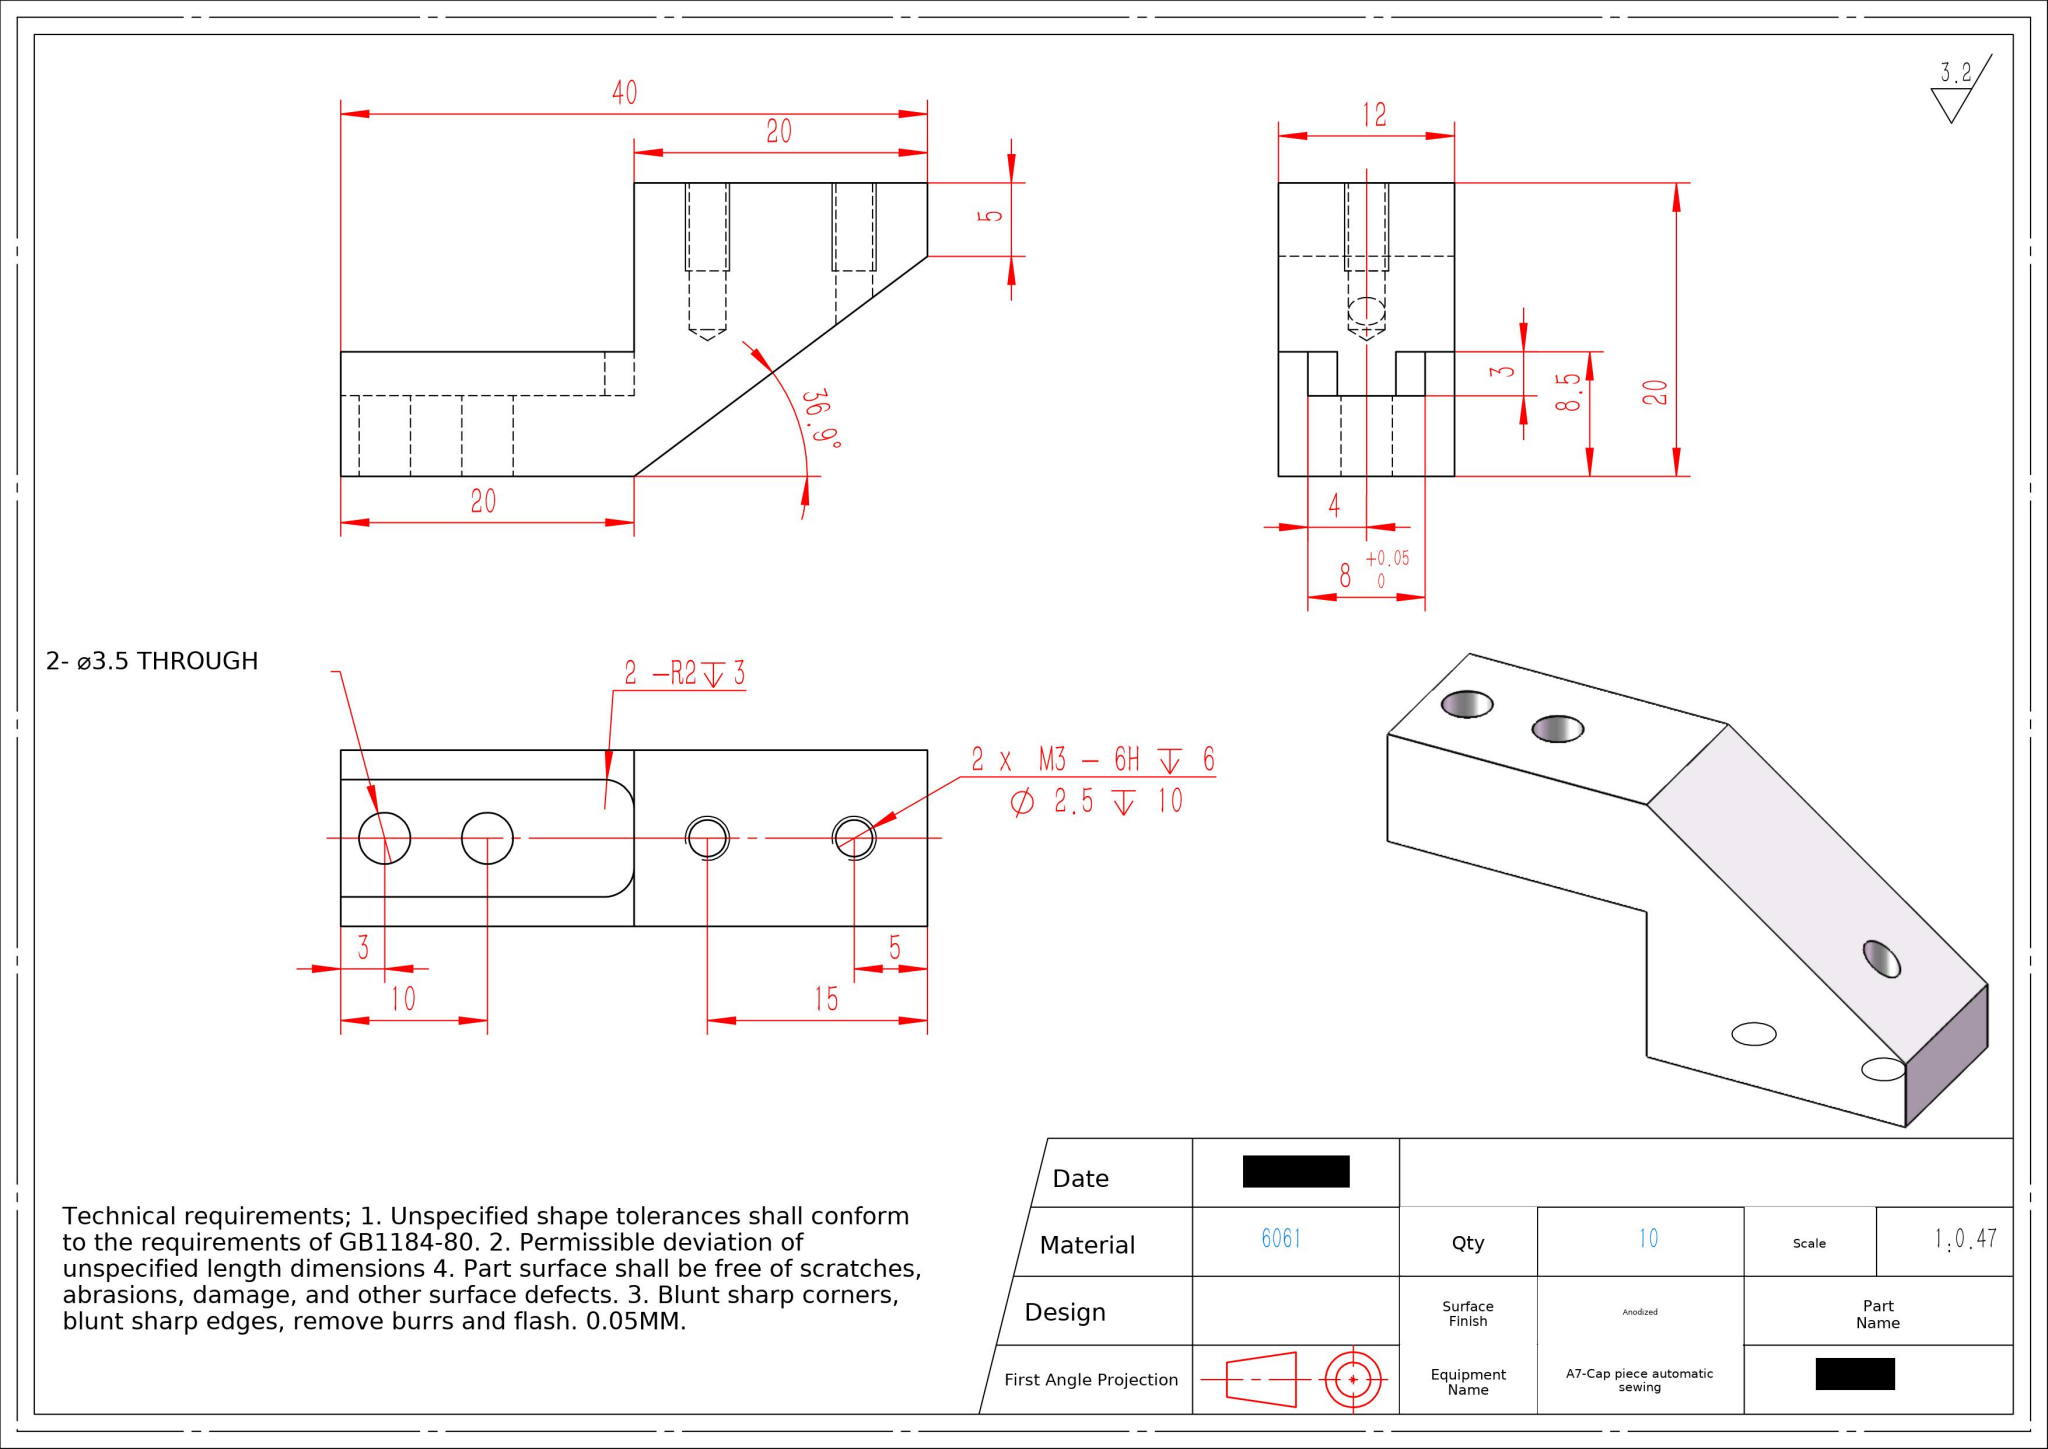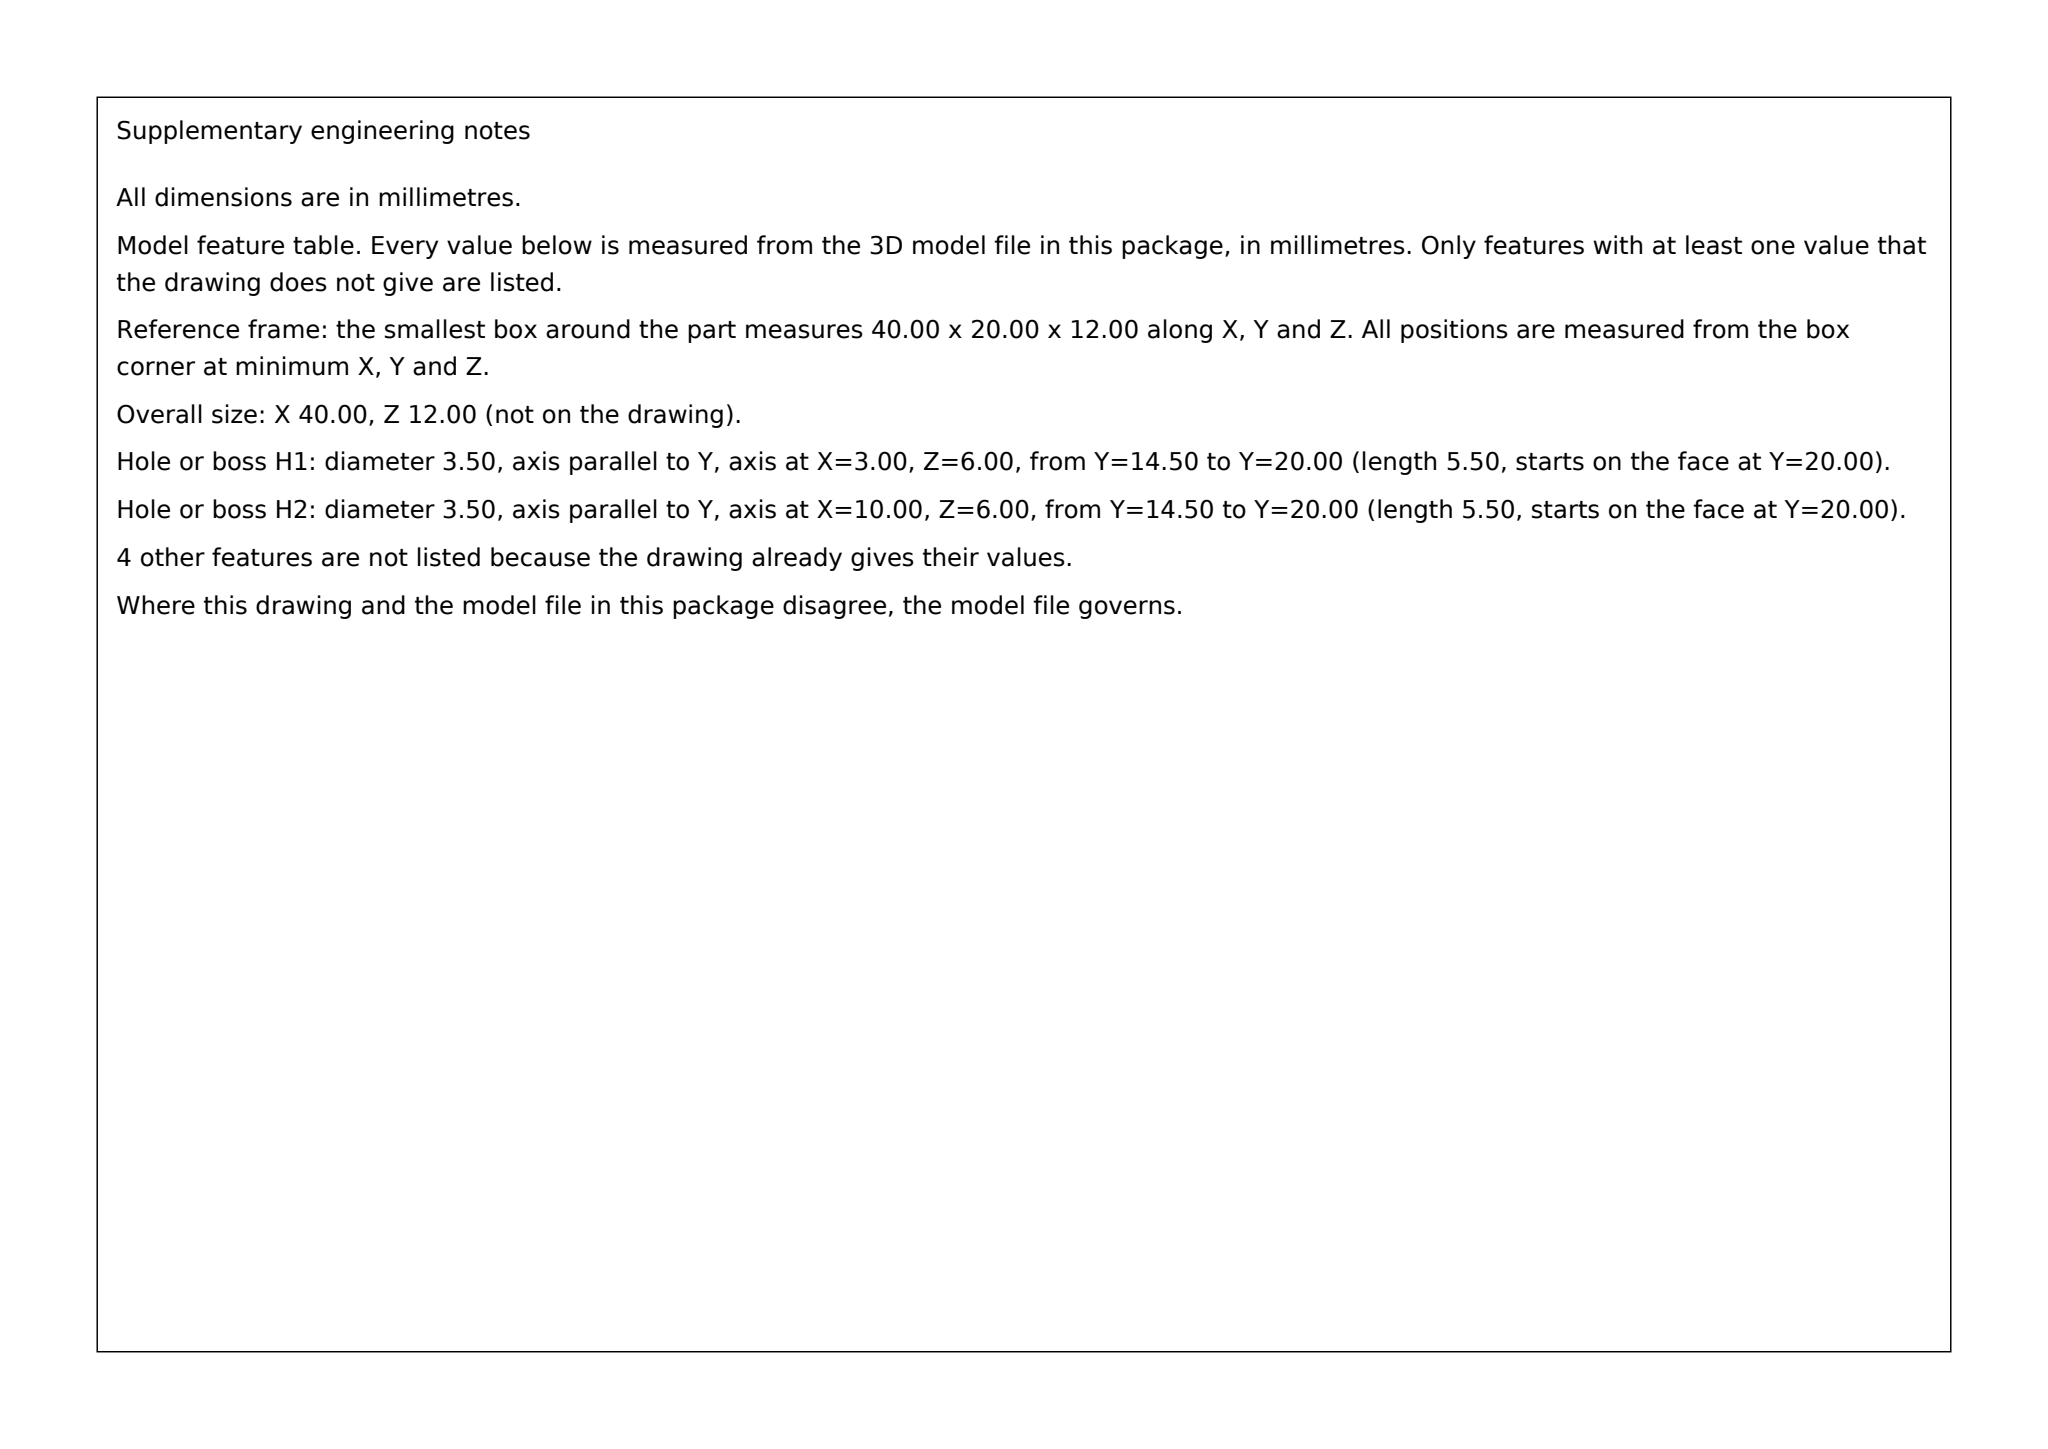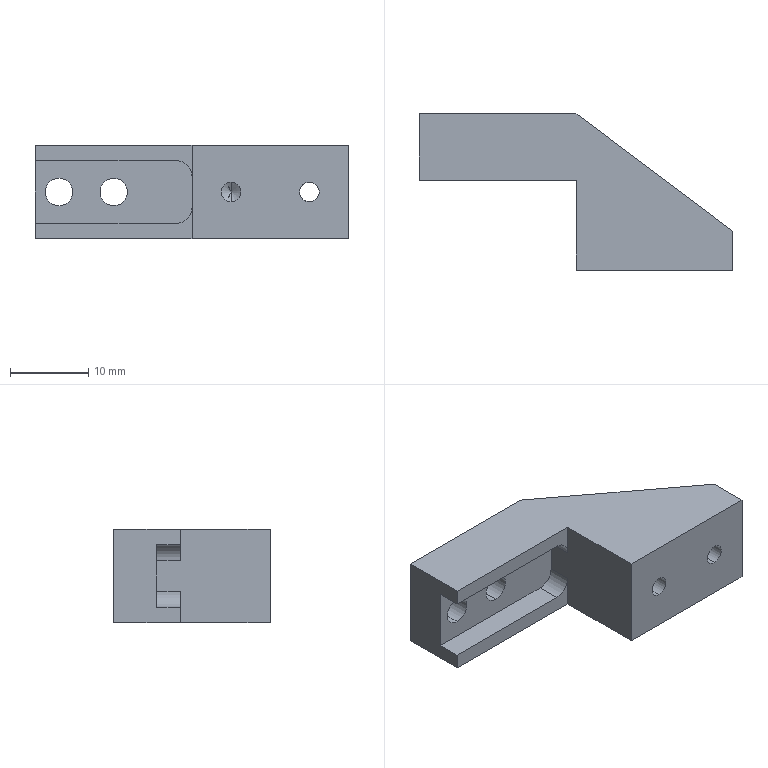Part | SolidWorks | mm | material 6061 | 1 solid | 25 faces | box 40 x 20 x 12 mm | volume 4366 mm3 | plane 13 | cylinder 10 | cone 2 | commonest cylinder face diameters 2.5 x4 3.5 x4 4 x2
build123d program:
from build123d import *

# Parameters (mm, degrees)
SKETCH1_W           = 40
SKETCH1_H           = 12
BOSS_EXTRUDE1_DEPTH = 20
SKETCH2_W           = 20
SKETCH2_H           = 11.5
CUT_EXTRUDE1_DEPTH  = 31.725
SKETCH3_W           = 20
SKETCH3_H           = 8
CUT_EXTRUDE2_DEPTH  = 3
SKETCH4_R           = 1.75
CUT_EXTRUDE3_DEPTH  = 29.914
FILLET1_R           = 2
LPATTERN1_COUNT     = 2
LPATTERN1_PITCH     = 10
CUT_EXTRUDE4_DEPTH  = 31.725


with BuildPart() as part:
    # Sketch1 → Boss-Extrude1 (new body)
    with BuildSketch(Plane(origin=(0, 0, 0), x_dir=(1, 0, 0), z_dir=(0, 1, 0))):
        Rectangle(SKETCH1_W, SKETCH1_H)
    extrude(amount=BOSS_EXTRUDE1_DEPTH)

    # Sketch2 → Cut-Extrude1 (cut, through all)
    with BuildSketch(Plane.XY.offset(6)):
        with Locations((-10, 5.75)):
            Rectangle(SKETCH2_W, SKETCH2_H)
    extrude(amount=-CUT_EXTRUDE1_DEPTH, mode=Mode.SUBTRACT)

    # Sketch3 → Cut-Extrude2 (cut)
    with BuildSketch(Plane(origin=(0, 11.5, 0), x_dir=(-1, 0, 0), z_dir=(0, -1, 0))):
        with Locations((10, 0)):
            Rectangle(SKETCH3_W, SKETCH3_H)
    extrude(amount=-CUT_EXTRUDE2_DEPTH, mode=Mode.SUBTRACT)

    # Sketch4 → Cut-Extrude3 (cut, through all)
    with BuildSketch(Plane(origin=(0, 20, 0), x_dir=(1, 0, 0), z_dir=(0, 1, 0))):
        with Locations(Location((-17, 0, 0), (0, 0, 270))):
            Circle(SKETCH4_R)
        with Locations(Location((-10, 0, 0), (0, 0, 270))):
            Circle(SKETCH4_R)
    extrude(amount=-CUT_EXTRUDE3_DEPTH, mode=Mode.SUBTRACT)

    # Fillet1
    fillet1_edges = [part.edges().sort_by_distance(p)[0] for p in [
        (0, 13, 4),
        (0, 13, -4),
    ]]
    fillet(fillet1_edges, radius=FILLET1_R)

    # Sketch5 → M3 Tapped Hole1 (revolve, cut)
    with BuildSketch(Plane(origin=(5, 0, 0), x_dir=(0, 0, -1), z_dir=(1, 0, 0))):
        Polygon((0, 0), (0, 10.751), (1.25, 10), (1.25, 0), align=None)
    m3_tapped_hole1 = revolve(axis=Axis((5, -6.35, 0), (0, 1, 0)), mode=Mode.SUBTRACT)

    # LPattern1: M3 Tapped Hole1 ×2
    with Locations(*[(i * LPATTERN1_PITCH, 0, 0) for i in range(1, LPATTERN1_COUNT)]):
        add(m3_tapped_hole1, mode=Mode.SUBTRACT)

    # Sketch6 → Cut-Extrude4 (cut, through all)
    with BuildSketch(Plane.XY.offset(6)):
        Polygon((20, 5), (0, 20), (20, 20), align=None)
    extrude(amount=-CUT_EXTRUDE4_DEPTH, mode=Mode.SUBTRACT)


solid = part.part
STEP:
#1=CARTESIAN_POINT('',(15.,8.75,-1.25));
#2=VERTEX_POINT('',#1);
#3=CARTESIAN_POINT('',(15.,8.75,1.25));
#4=VERTEX_POINT('',#3);
#5=CARTESIAN_POINT('',(15.,8.75,-1.25));
#6=CARTESIAN_POINT('',(12.5,10.625,-1.25));
#7=CARTESIAN_POINT('',(12.5,10.625,1.25));
#8=CARTESIAN_POINT('',(15.,8.75,1.25));
#9=(BOUNDED_CURVE()B_SPLINE_CURVE(3,(#5,#6,#7,#8),.UNSPECIFIED.,.F.,.T.)B_SPLINE_CURVE_WITH_KNOTS((4,4),(1.571,4.712),.UNSPECIFIED.)CURVE()GEOMETRIC_REPRESENTATION_ITEM()RATIONAL_B_SPLINE_CURVE((1.,0.3333,0.3333,1.))REPRESENTATION_ITEM(''));
#10=EDGE_CURVE('',#2,#4,#9,.T.);
#11=ORIENTED_EDGE('',*,*,#10,.T.);
#12=CARTESIAN_POINT('',(15.,-0.,1.25));
#13=VERTEX_POINT('',#12);
#14=CARTESIAN_POINT('',(15.,0.,1.25));
#15=DIRECTION('',(0.,-1.,0.));
#16=VECTOR('',#15,1000.);
#17=LINE('',#14,#16);
#18=EDGE_CURVE('',#4,#13,#17,.T.);
#19=ORIENTED_EDGE('',*,*,#18,.T.);
#20=CARTESIAN_POINT('',(15.,-0.,-1.25));
#21=VERTEX_POINT('',#20);
#22=CARTESIAN_POINT('',(15.,-0.,0.));
#23=DIRECTION('',(0.,-1.,0.));
#24=DIRECTION('',(0.,0.,-1.));
#25=AXIS2_PLACEMENT_3D('',#22,#23,#24);
#26=CIRCLE('',#25,1.25);
#27=EDGE_CURVE('',#13,#21,#26,.T.);
#28=ORIENTED_EDGE('',*,*,#27,.T.);
#29=CARTESIAN_POINT('',(15.,0.,-1.25));
#30=DIRECTION('',(0.,-1.,0.));
#31=VECTOR('',#30,1000.);
#32=LINE('',#29,#31);
#33=EDGE_CURVE('',#2,#21,#32,.T.);
#34=ORIENTED_EDGE('',*,*,#33,.F.);
#35=EDGE_LOOP('',(#11,#19,#28,#34));
#36=FACE_OUTER_BOUND('',#35,.T.);
#37=CARTESIAN_POINT('',(15.,0.,0.));
#38=DIRECTION('',(0.,-1.,0.));
#39=DIRECTION('',(0.,0.,-1.));
#40=AXIS2_PLACEMENT_3D('',#37,#38,#39);
#41=CYLINDRICAL_SURFACE('',#40,1.25);
#42=ADVANCED_FACE('',(#36),#41,.F.);
#43=CARTESIAN_POINT('',(5.,10.,1.25));
#44=VERTEX_POINT('',#43);
#45=CARTESIAN_POINT('',(5.,10.,-1.25));
#46=VERTEX_POINT('',#45);
#47=CARTESIAN_POINT('',(5.,10.,0.));
#48=DIRECTION('',(0.,-1.,0.));
#49=DIRECTION('',(0.,0.,-1.));
#50=AXIS2_PLACEMENT_3D('',#47,#48,#49);
#51=CIRCLE('',#50,1.25);
#52=EDGE_CURVE('',#44,#46,#51,.T.);
#53=ORIENTED_EDGE('',*,*,#52,.F.);
#54=CARTESIAN_POINT('',(5.,-0.,1.25));
#55=VERTEX_POINT('',#54);
#56=CARTESIAN_POINT('',(5.,0.,1.25));
#57=DIRECTION('',(0.,-1.,0.));
#58=VECTOR('',#57,1000.);
#59=LINE('',#56,#58);
#60=EDGE_CURVE('',#44,#55,#59,.T.);
#61=ORIENTED_EDGE('',*,*,#60,.T.);
#62=CARTESIAN_POINT('',(5.,-0.,-1.25));
#63=VERTEX_POINT('',#62);
#64=CARTESIAN_POINT('',(5.,-0.,0.));
#65=DIRECTION('',(0.,-1.,0.));
#66=DIRECTION('',(0.,0.,-1.));
#67=AXIS2_PLACEMENT_3D('',#64,#65,#66);
#68=CIRCLE('',#67,1.25);
#69=EDGE_CURVE('',#55,#63,#68,.T.);
#70=ORIENTED_EDGE('',*,*,#69,.T.);
#71=CARTESIAN_POINT('',(5.,0.,-1.25));
#72=DIRECTION('',(0.,-1.,0.));
#73=VECTOR('',#72,1000.);
#74=LINE('',#71,#73);
#75=EDGE_CURVE('',#46,#63,#74,.T.);
#76=ORIENTED_EDGE('',*,*,#75,.F.);
#77=EDGE_LOOP('',(#53,#61,#70,#76));
#78=FACE_OUTER_BOUND('',#77,.T.);
#79=CARTESIAN_POINT('',(5.,0.,0.));
#80=DIRECTION('',(0.,-1.,0.));
#81=DIRECTION('',(0.,0.,-1.));
#82=AXIS2_PLACEMENT_3D('',#79,#80,#81);
#83=CYLINDRICAL_SURFACE('',#82,1.25);
#84=ADVANCED_FACE('',(#78),#83,.F.);
#85=CARTESIAN_POINT('',(5.,10.751,0.));
#86=VERTEX_POINT('',#85);
#87=CARTESIAN_POINT('',(5.,10.,-1.25));
#88=DIRECTION('',(0.,-0.515,-0.8572));
#89=VECTOR('',#88,1000.);
#90=LINE('',#87,#89);
#91=EDGE_CURVE('',#86,#46,#90,.T.);
#92=ORIENTED_EDGE('',*,*,#91,.F.);
#93=CARTESIAN_POINT('',(5.,10.,1.25));
#94=DIRECTION('',(0.,-0.515,0.8572));
#95=VECTOR('',#94,1000.);
#96=LINE('',#93,#95);
#97=EDGE_CURVE('',#86,#44,#96,.T.);
#98=ORIENTED_EDGE('',*,*,#97,.T.);
#99=ORIENTED_EDGE('',*,*,#52,.T.);
#100=EDGE_LOOP('',(#92,#98,#99));
#101=FACE_OUTER_BOUND('',#100,.T.);
#102=CARTESIAN_POINT('',(5.,10.,0.));
#103=DIRECTION('',(0.,-1.,0.));
#104=DIRECTION('',(0.,0.,-1.));
#105=AXIS2_PLACEMENT_3D('',#102,#103,#104);
#106=CONICAL_SURFACE('',#105,1.25,1.03);
#107=ADVANCED_FACE('',(#101),#106,.F.);
#108=CARTESIAN_POINT('',(-17.,14.5,1.75));
#109=VERTEX_POINT('',#108);
#110=CARTESIAN_POINT('',(-17.,14.5,-1.75));
#111=VERTEX_POINT('',#110);
#112=CARTESIAN_POINT('',(-17.,14.5,0.));
#113=DIRECTION('',(0.,-1.,0.));
#114=DIRECTION('',(0.,0.,-1.));
#115=AXIS2_PLACEMENT_3D('',#112,#113,#114);
#116=CIRCLE('',#115,1.75);
#117=EDGE_CURVE('',#109,#111,#116,.T.);
#118=ORIENTED_EDGE('',*,*,#117,.T.);
#119=CARTESIAN_POINT('',(-17.,20.,-1.75));
#120=VERTEX_POINT('',#119);
#121=CARTESIAN_POINT('',(-17.,0.,-1.75));
#122=DIRECTION('',(0.,1.,0.));
#123=VECTOR('',#122,1000.);
#124=LINE('',#121,#123);
#125=EDGE_CURVE('',#111,#120,#124,.T.);
#126=ORIENTED_EDGE('',*,*,#125,.T.);
#127=CARTESIAN_POINT('',(-17.,20.,1.75));
#128=VERTEX_POINT('',#127);
#129=CARTESIAN_POINT('',(-17.,20.,0.));
#130=DIRECTION('',(0.,1.,0.));
#131=DIRECTION('',(0.,0.,1.));
#132=AXIS2_PLACEMENT_3D('',#129,#130,#131);
#133=CIRCLE('',#132,1.75);
#134=EDGE_CURVE('',#120,#128,#133,.T.);
#135=ORIENTED_EDGE('',*,*,#134,.T.);
#136=CARTESIAN_POINT('',(-17.,0.,1.75));
#137=DIRECTION('',(0.,1.,0.));
#138=VECTOR('',#137,1000.);
#139=LINE('',#136,#138);
#140=EDGE_CURVE('',#109,#128,#139,.T.);
#141=ORIENTED_EDGE('',*,*,#140,.F.);
#142=EDGE_LOOP('',(#118,#126,#135,#141));
#143=FACE_OUTER_BOUND('',#142,.T.);
#144=CARTESIAN_POINT('',(-17.,0.,0.));
#145=DIRECTION('',(0.,1.,0.));
#146=DIRECTION('',(0.,0.,1.));
#147=AXIS2_PLACEMENT_3D('',#144,#145,#146);
#148=CYLINDRICAL_SURFACE('',#147,1.75);
#149=ADVANCED_FACE('',(#143),#148,.F.);
#150=CARTESIAN_POINT('',(-10.,14.5,1.75));
#151=VERTEX_POINT('',#150);
#152=CARTESIAN_POINT('',(-10.,14.5,-1.75));
#153=VERTEX_POINT('',#152);
#154=CARTESIAN_POINT('',(-10.,14.5,0.));
#155=DIRECTION('',(0.,-1.,0.));
#156=DIRECTION('',(0.,0.,-1.));
#157=AXIS2_PLACEMENT_3D('',#154,#155,#156);
#158=CIRCLE('',#157,1.75);
#159=EDGE_CURVE('',#151,#153,#158,.T.);
#160=ORIENTED_EDGE('',*,*,#159,.T.);
#161=CARTESIAN_POINT('',(-10.,20.,-1.75));
#162=VERTEX_POINT('',#161);
#163=CARTESIAN_POINT('',(-10.,0.,-1.75));
#164=DIRECTION('',(0.,1.,0.));
#165=VECTOR('',#164,1000.);
#166=LINE('',#163,#165);
#167=EDGE_CURVE('',#153,#162,#166,.T.);
#168=ORIENTED_EDGE('',*,*,#167,.T.);
#169=CARTESIAN_POINT('',(-10.,20.,1.75));
#170=VERTEX_POINT('',#169);
#171=CARTESIAN_POINT('',(-10.,20.,0.));
#172=DIRECTION('',(0.,1.,0.));
#173=DIRECTION('',(0.,0.,1.));
#174=AXIS2_PLACEMENT_3D('',#171,#172,#173);
#175=CIRCLE('',#174,1.75);
#176=EDGE_CURVE('',#162,#170,#175,.T.);
#177=ORIENTED_EDGE('',*,*,#176,.T.);
#178=CARTESIAN_POINT('',(-10.,0.,1.75));
#179=DIRECTION('',(0.,1.,0.));
#180=VECTOR('',#179,1000.);
#181=LINE('',#178,#180);
#182=EDGE_CURVE('',#151,#170,#181,.T.);
#183=ORIENTED_EDGE('',*,*,#182,.F.);
#184=EDGE_LOOP('',(#160,#168,#177,#183));
#185=FACE_OUTER_BOUND('',#184,.T.);
#186=CARTESIAN_POINT('',(-10.,0.,0.));
#187=DIRECTION('',(0.,1.,0.));
#188=DIRECTION('',(0.,0.,1.));
#189=AXIS2_PLACEMENT_3D('',#186,#187,#188);
#190=CYLINDRICAL_SURFACE('',#189,1.75);
#191=ADVANCED_FACE('',(#185),#190,.F.);
#192=CARTESIAN_POINT('',(0.,11.5,-6.));
#193=VERTEX_POINT('',#192);
#194=CARTESIAN_POINT('',(0.,11.5,-2.));
#195=VERTEX_POINT('',#194);
#196=CARTESIAN_POINT('',(0.,11.5,-6.));
#197=DIRECTION('',(0.,0.,1.));
#198=VECTOR('',#197,1000.);
#199=LINE('',#196,#198);
#200=EDGE_CURVE('',#193,#195,#199,.T.);
#201=ORIENTED_EDGE('',*,*,#200,.T.);
#202=CARTESIAN_POINT('',(-2.,11.5,-4.));
#203=VERTEX_POINT('',#202);
#204=CARTESIAN_POINT('',(-2.,11.5,-2.));
#205=DIRECTION('',(0.,1.,0.));
#206=DIRECTION('',(0.,0.,1.));
#207=AXIS2_PLACEMENT_3D('',#204,#205,#206);
#208=CIRCLE('',#207,2.);
#209=EDGE_CURVE('',#195,#203,#208,.T.);
#210=ORIENTED_EDGE('',*,*,#209,.T.);
#211=CARTESIAN_POINT('',(-20.,11.5,-4.));
#212=VERTEX_POINT('',#211);
#213=CARTESIAN_POINT('',(-20.,11.5,-4.));
#214=DIRECTION('',(1.,0.,0.));
#215=VECTOR('',#214,1000.);
#216=LINE('',#213,#215);
#217=EDGE_CURVE('',#212,#203,#216,.T.);
#218=ORIENTED_EDGE('',*,*,#217,.F.);
#219=CARTESIAN_POINT('',(-20.,11.5,-6.));
#220=VERTEX_POINT('',#219);
#221=CARTESIAN_POINT('',(-20.,11.5,-6.));
#222=DIRECTION('',(0.,0.,1.));
#223=VECTOR('',#222,1000.);
#224=LINE('',#221,#223);
#225=EDGE_CURVE('',#220,#212,#224,.T.);
#226=ORIENTED_EDGE('',*,*,#225,.F.);
#227=CARTESIAN_POINT('',(-20.,11.5,-6.));
#228=DIRECTION('',(-1.,0.,0.));
#229=VECTOR('',#228,1000.);
#230=LINE('',#227,#229);
#231=EDGE_CURVE('',#193,#220,#230,.T.);
#232=ORIENTED_EDGE('',*,*,#231,.F.);
#233=EDGE_LOOP('',(#201,#210,#218,#226,#232));
#234=FACE_OUTER_BOUND('',#233,.T.);
#235=CARTESIAN_POINT('',(-20.,11.5,-6.));
#236=DIRECTION('',(0.,1.,0.));
#237=DIRECTION('',(0.,0.,1.));
#238=AXIS2_PLACEMENT_3D('',#235,#236,#237);
#239=PLANE('',#238);
#240=ADVANCED_FACE('',(#234),#239,.F.);
#241=CARTESIAN_POINT('',(20.,5.,-6.));
#242=VERTEX_POINT('',#241);
#243=CARTESIAN_POINT('',(20.,0.,-6.));
#244=VERTEX_POINT('',#243);
#245=CARTESIAN_POINT('',(20.,20.,-6.));
#246=DIRECTION('',(0.,-1.,0.));
#247=VECTOR('',#246,1000.);
#248=LINE('',#245,#247);
#249=EDGE_CURVE('',#242,#244,#248,.T.);
#250=ORIENTED_EDGE('',*,*,#249,.F.);
#251=CARTESIAN_POINT('',(20.,5.,6.));
#252=VERTEX_POINT('',#251);
#253=CARTESIAN_POINT('',(20.,5.,-6.));
#254=DIRECTION('',(0.,0.,1.));
#255=VECTOR('',#254,1000.);
#256=LINE('',#253,#255);
#257=EDGE_CURVE('',#242,#252,#256,.T.);
#258=ORIENTED_EDGE('',*,*,#257,.T.);
#259=CARTESIAN_POINT('',(20.,0.,6.));
#260=VERTEX_POINT('',#259);
#261=CARTESIAN_POINT('',(20.,20.,6.));
#262=DIRECTION('',(0.,-1.,0.));
#263=VECTOR('',#262,1000.);
#264=LINE('',#261,#263);
#265=EDGE_CURVE('',#252,#260,#264,.T.);
#266=ORIENTED_EDGE('',*,*,#265,.T.);
#267=CARTESIAN_POINT('',(20.,0.,-6.));
#268=DIRECTION('',(0.,0.,-1.));
#269=VECTOR('',#268,1000.);
#270=LINE('',#267,#269);
#271=EDGE_CURVE('',#260,#244,#270,.T.);
#272=ORIENTED_EDGE('',*,*,#271,.T.);
#273=EDGE_LOOP('',(#250,#258,#266,#272));
#274=FACE_OUTER_BOUND('',#273,.T.);
#275=CARTESIAN_POINT('',(20.,20.,-6.));
#276=DIRECTION('',(-1.,0.,0.));
#277=DIRECTION('',(0.,0.,1.));
#278=AXIS2_PLACEMENT_3D('',#275,#276,#277);
#279=PLANE('',#278);
#280=ADVANCED_FACE('',(#274),#279,.F.);
#281=CARTESIAN_POINT('',(-0.,20.,-6.));
#282=VERTEX_POINT('',#281);
#283=CARTESIAN_POINT('',(-20.,20.,-6.));
#284=VERTEX_POINT('',#283);
#285=CARTESIAN_POINT('',(-20.,20.,-6.));
#286=DIRECTION('',(-1.,0.,0.));
#287=VECTOR('',#286,1000.);
#288=LINE('',#285,#287);
#289=EDGE_CURVE('',#282,#284,#288,.T.);
#290=ORIENTED_EDGE('',*,*,#289,.F.);
#291=CARTESIAN_POINT('',(20.,5.,-6.));
#292=DIRECTION('',(0.8,-0.6,0.));
#293=VECTOR('',#292,1000.);
#294=LINE('',#291,#293);
#295=EDGE_CURVE('',#282,#242,#294,.T.);
#296=ORIENTED_EDGE('',*,*,#295,.T.);
#297=ORIENTED_EDGE('',*,*,#249,.T.);
#298=CARTESIAN_POINT('',(0.,0.,-6.));
#299=VERTEX_POINT('',#298);
#300=CARTESIAN_POINT('',(-20.,0.,-6.));
#301=DIRECTION('',(-1.,0.,0.));
#302=VECTOR('',#301,1000.);
#303=LINE('',#300,#302);
#304=EDGE_CURVE('',#244,#299,#303,.T.);
#305=ORIENTED_EDGE('',*,*,#304,.T.);
#306=CARTESIAN_POINT('',(0.,0.,-6.));
#307=DIRECTION('',(0.,1.,0.));
#308=VECTOR('',#307,1000.);
#309=LINE('',#306,#308);
#310=EDGE_CURVE('',#299,#193,#309,.T.);
#311=ORIENTED_EDGE('',*,*,#310,.T.);
#312=ORIENTED_EDGE('',*,*,#231,.T.);
#313=CARTESIAN_POINT('',(-20.,20.,-6.));
#314=DIRECTION('',(0.,-1.,0.));
#315=VECTOR('',#314,1000.);
#316=LINE('',#313,#315);
#317=EDGE_CURVE('',#284,#220,#316,.T.);
#318=ORIENTED_EDGE('',*,*,#317,.F.);
#319=EDGE_LOOP('',(#290,#296,#297,#305,#311,#312,#318));
#320=FACE_OUTER_BOUND('',#319,.T.);
#321=CARTESIAN_POINT('',(-20.,20.,-6.));
#322=DIRECTION('',(0.,0.,1.));
#323=DIRECTION('',(1.,0.,0.));
#324=AXIS2_PLACEMENT_3D('',#321,#322,#323);
#325=PLANE('',#324);
#326=ADVANCED_FACE('',(#320),#325,.F.);
#327=ORIENTED_EDGE('',*,*,#225,.T.);
#328=CARTESIAN_POINT('',(-20.,14.5,-4.));
#329=VERTEX_POINT('',#328);
#330=CARTESIAN_POINT('',(-20.,14.5,-4.));
#331=DIRECTION('',(0.,-1.,0.));
#332=VECTOR('',#331,1000.);
#333=LINE('',#330,#332);
#334=EDGE_CURVE('',#329,#212,#333,.T.);
#335=ORIENTED_EDGE('',*,*,#334,.F.);
#336=CARTESIAN_POINT('',(-20.,14.5,4.));
#337=VERTEX_POINT('',#336);
#338=CARTESIAN_POINT('',(-20.,14.5,4.));
#339=DIRECTION('',(0.,0.,-1.));
#340=VECTOR('',#339,1000.);
#341=LINE('',#338,#340);
#342=EDGE_CURVE('',#337,#329,#341,.T.);
#343=ORIENTED_EDGE('',*,*,#342,.F.);
#344=CARTESIAN_POINT('',(-20.,11.5,4.));
#345=VERTEX_POINT('',#344);
#346=CARTESIAN_POINT('',(-20.,14.5,4.));
#347=DIRECTION('',(0.,-1.,0.));
#348=VECTOR('',#347,1000.);
#349=LINE('',#346,#348);
#350=EDGE_CURVE('',#337,#345,#349,.T.);
#351=ORIENTED_EDGE('',*,*,#350,.T.);
#352=CARTESIAN_POINT('',(-20.,11.5,6.));
#353=VERTEX_POINT('',#352);
#354=CARTESIAN_POINT('',(-20.,11.5,-6.));
#355=DIRECTION('',(0.,0.,1.));
#356=VECTOR('',#355,1000.);
#357=LINE('',#354,#356);
#358=EDGE_CURVE('',#345,#353,#357,.T.);
#359=ORIENTED_EDGE('',*,*,#358,.T.);
#360=CARTESIAN_POINT('',(-20.,20.,6.));
#361=VERTEX_POINT('',#360);
#362=CARTESIAN_POINT('',(-20.,20.,6.));
#363=DIRECTION('',(0.,-1.,0.));
#364=VECTOR('',#363,1000.);
#365=LINE('',#362,#364);
#366=EDGE_CURVE('',#361,#353,#365,.T.);
#367=ORIENTED_EDGE('',*,*,#366,.F.);
#368=CARTESIAN_POINT('',(-20.,20.,-6.));
#369=DIRECTION('',(0.,0.,1.));
#370=VECTOR('',#369,1000.);
#371=LINE('',#368,#370);
#372=EDGE_CURVE('',#284,#361,#371,.T.);
#373=ORIENTED_EDGE('',*,*,#372,.F.);
#374=ORIENTED_EDGE('',*,*,#317,.T.);
#375=EDGE_LOOP('',(#327,#335,#343,#351,#359,#367,#373,#374));
#376=FACE_OUTER_BOUND('',#375,.T.);
#377=CARTESIAN_POINT('',(-20.,20.,-6.));
#378=DIRECTION('',(1.,0.,0.));
#379=DIRECTION('',(0.,0.,-1.));
#380=AXIS2_PLACEMENT_3D('',#377,#378,#379);
#381=PLANE('',#380);
#382=ADVANCED_FACE('',(#376),#381,.F.);
#383=ORIENTED_EDGE('',*,*,#265,.F.);
#384=CARTESIAN_POINT('',(-0.,20.,6.));
#385=VERTEX_POINT('',#384);
#386=CARTESIAN_POINT('',(20.,5.,6.));
#387=DIRECTION('',(0.8,-0.6,0.));
#388=VECTOR('',#387,1000.);
#389=LINE('',#386,#388);
#390=EDGE_CURVE('',#385,#252,#389,.T.);
#391=ORIENTED_EDGE('',*,*,#390,.F.);
#392=CARTESIAN_POINT('',(-20.,20.,6.));
#393=DIRECTION('',(1.,0.,0.));
#394=VECTOR('',#393,1000.);
#395=LINE('',#392,#394);
#396=EDGE_CURVE('',#361,#385,#395,.T.);
#397=ORIENTED_EDGE('',*,*,#396,.F.);
#398=ORIENTED_EDGE('',*,*,#366,.T.);
#399=CARTESIAN_POINT('',(0.,11.5,6.));
#400=VERTEX_POINT('',#399);
#401=CARTESIAN_POINT('',(-20.,11.5,6.));
#402=DIRECTION('',(-1.,0.,0.));
#403=VECTOR('',#402,1000.);
#404=LINE('',#401,#403);
#405=EDGE_CURVE('',#400,#353,#404,.T.);
#406=ORIENTED_EDGE('',*,*,#405,.F.);
#407=CARTESIAN_POINT('',(0.,0.,6.));
#408=VERTEX_POINT('',#407);
#409=CARTESIAN_POINT('',(0.,0.,6.));
#410=DIRECTION('',(0.,1.,0.));
#411=VECTOR('',#410,1000.);
#412=LINE('',#409,#411);
#413=EDGE_CURVE('',#408,#400,#412,.T.);
#414=ORIENTED_EDGE('',*,*,#413,.F.);
#415=CARTESIAN_POINT('',(-20.,0.,6.));
#416=DIRECTION('',(1.,0.,0.));
#417=VECTOR('',#416,1000.);
#418=LINE('',#415,#417);
#419=EDGE_CURVE('',#408,#260,#418,.T.);
#420=ORIENTED_EDGE('',*,*,#419,.T.);
#421=EDGE_LOOP('',(#383,#391,#397,#398,#406,#414,#420));
#422=FACE_OUTER_BOUND('',#421,.T.);
#423=CARTESIAN_POINT('',(-20.,20.,6.));
#424=DIRECTION('',(0.,0.,-1.));
#425=DIRECTION('',(-1.,0.,0.));
#426=AXIS2_PLACEMENT_3D('',#423,#424,#425);
#427=PLANE('',#426);
#428=ADVANCED_FACE('',(#422),#427,.F.);
#429=CARTESIAN_POINT('',(-0.,20.,-6.));
#430=DIRECTION('',(0.,0.,1.));
#431=VECTOR('',#430,1000.);
#432=LINE('',#429,#431);
#433=EDGE_CURVE('',#282,#385,#432,.T.);
#434=ORIENTED_EDGE('',*,*,#433,.F.);
#435=ORIENTED_EDGE('',*,*,#289,.T.);
#436=ORIENTED_EDGE('',*,*,#372,.T.);
#437=ORIENTED_EDGE('',*,*,#396,.T.);
#438=EDGE_LOOP('',(#434,#435,#436,#437));
#439=FACE_OUTER_BOUND('',#438,.T.);
#440=CARTESIAN_POINT('',(-17.,20.,0.));
#441=DIRECTION('',(0.,1.,0.));
#442=DIRECTION('',(0.,0.,1.));
#443=AXIS2_PLACEMENT_3D('',#440,#441,#442);
#444=CIRCLE('',#443,1.75);
#445=EDGE_CURVE('',#128,#120,#444,.T.);
#446=ORIENTED_EDGE('',*,*,#445,.F.);
#447=ORIENTED_EDGE('',*,*,#134,.F.);
#448=EDGE_LOOP('',(#446,#447));
#449=FACE_BOUND('',#448,.T.);
#450=CARTESIAN_POINT('',(-10.,20.,0.));
#451=DIRECTION('',(0.,1.,0.));
#452=DIRECTION('',(0.,0.,1.));
#453=AXIS2_PLACEMENT_3D('',#450,#451,#452);
#454=CIRCLE('',#453,1.75);
#455=EDGE_CURVE('',#170,#162,#454,.T.);
#456=ORIENTED_EDGE('',*,*,#455,.F.);
#457=ORIENTED_EDGE('',*,*,#176,.F.);
#458=EDGE_LOOP('',(#456,#457));
#459=FACE_BOUND('',#458,.T.);
#460=CARTESIAN_POINT('',(0.,20.,0.));
#461=DIRECTION('',(0.,1.,0.));
#462=DIRECTION('',(0.,0.,1.));
#463=AXIS2_PLACEMENT_3D('',#460,#461,#462);
#464=PLANE('',#463);
#465=ADVANCED_FACE('',(#439,#449,#459),#464,.T.);
#466=CARTESIAN_POINT('',(15.,-0.,0.));
#467=DIRECTION('',(0.,-1.,0.));
#468=DIRECTION('',(0.,0.,-1.));
#469=AXIS2_PLACEMENT_3D('',#466,#467,#468);
#470=CIRCLE('',#469,1.25);
#471=EDGE_CURVE('',#21,#13,#470,.T.);
#472=ORIENTED_EDGE('',*,*,#471,.F.);
#473=ORIENTED_EDGE('',*,*,#27,.F.);
#474=EDGE_LOOP('',(#472,#473));
#475=FACE_BOUND('',#474,.T.);
#476=CARTESIAN_POINT('',(5.,-0.,0.));
#477=DIRECTION('',(0.,-1.,0.));
#478=DIRECTION('',(0.,0.,-1.));
#479=AXIS2_PLACEMENT_3D('',#476,#477,#478);
#480=CIRCLE('',#479,1.25);
#481=EDGE_CURVE('',#63,#55,#480,.T.);
#482=ORIENTED_EDGE('',*,*,#481,.F.);
#483=ORIENTED_EDGE('',*,*,#69,.F.);
#484=EDGE_LOOP('',(#482,#483));
#485=FACE_BOUND('',#484,.T.);
#486=ORIENTED_EDGE('',*,*,#419,.F.);
#487=CARTESIAN_POINT('',(0.,0.,-6.));
#488=DIRECTION('',(0.,0.,1.));
#489=VECTOR('',#488,1000.);
#490=LINE('',#487,#489);
#491=EDGE_CURVE('',#299,#408,#490,.T.);
#492=ORIENTED_EDGE('',*,*,#491,.F.);
#493=ORIENTED_EDGE('',*,*,#304,.F.);
#494=ORIENTED_EDGE('',*,*,#271,.F.);
#495=EDGE_LOOP('',(#486,#492,#493,#494));
#496=FACE_OUTER_BOUND('',#495,.T.);
#497=CARTESIAN_POINT('',(0.,0.,0.));
#498=DIRECTION('',(0.,1.,0.));
#499=DIRECTION('',(0.,0.,1.));
#500=AXIS2_PLACEMENT_3D('',#497,#498,#499);
#501=PLANE('',#500);
#502=ADVANCED_FACE('',(#475,#485,#496),#501,.F.);
#503=ORIENTED_EDGE('',*,*,#358,.F.);
#504=CARTESIAN_POINT('',(-2.,11.5,4.));
#505=VERTEX_POINT('',#504);
#506=CARTESIAN_POINT('',(-20.,11.5,4.));
#507=DIRECTION('',(-1.,0.,0.));
#508=VECTOR('',#507,1000.);
#509=LINE('',#506,#508);
#510=EDGE_CURVE('',#505,#345,#509,.T.);
#511=ORIENTED_EDGE('',*,*,#510,.F.);
#512=CARTESIAN_POINT('',(0.,11.5,2.));
#513=VERTEX_POINT('',#512);
#514=CARTESIAN_POINT('',(-2.,11.5,2.));
#515=DIRECTION('',(0.,1.,0.));
#516=DIRECTION('',(0.,0.,1.));
#517=AXIS2_PLACEMENT_3D('',#514,#515,#516);
#518=CIRCLE('',#517,2.);
#519=EDGE_CURVE('',#505,#513,#518,.T.);
#520=ORIENTED_EDGE('',*,*,#519,.T.);
#521=CARTESIAN_POINT('',(0.,11.5,-6.));
#522=DIRECTION('',(0.,0.,1.));
#523=VECTOR('',#522,1000.);
#524=LINE('',#521,#523);
#525=EDGE_CURVE('',#513,#400,#524,.T.);
#526=ORIENTED_EDGE('',*,*,#525,.T.);
#527=ORIENTED_EDGE('',*,*,#405,.T.);
#528=EDGE_LOOP('',(#503,#511,#520,#526,#527));
#529=FACE_OUTER_BOUND('',#528,.T.);
#530=CARTESIAN_POINT('',(-20.,11.5,-6.));
#531=DIRECTION('',(0.,1.,0.));
#532=DIRECTION('',(0.,0.,1.));
#533=AXIS2_PLACEMENT_3D('',#530,#531,#532);
#534=PLANE('',#533);
#535=ADVANCED_FACE('',(#529),#534,.F.);
#536=CARTESIAN_POINT('',(0.,14.5,-2.));
#537=VERTEX_POINT('',#536);
#538=CARTESIAN_POINT('',(0.,14.5,2.));
#539=VERTEX_POINT('',#538);
#540=CARTESIAN_POINT('',(0.,14.5,4.));
#541=DIRECTION('',(0.,0.,1.));
#542=VECTOR('',#541,1000.);
#543=LINE('',#540,#542);
#544=EDGE_CURVE('',#537,#539,#543,.T.);
#545=ORIENTED_EDGE('',*,*,#544,.F.);
#546=CARTESIAN_POINT('',(0.,11.5,-2.));
#547=DIRECTION('',(0.,-1.,0.));
#548=VECTOR('',#547,1000.);
#549=LINE('',#546,#548);
#550=EDGE_CURVE('',#537,#195,#549,.T.);
#551=ORIENTED_EDGE('',*,*,#550,.T.);
#552=ORIENTED_EDGE('',*,*,#200,.F.);
#553=ORIENTED_EDGE('',*,*,#310,.F.);
#554=ORIENTED_EDGE('',*,*,#491,.T.);
#555=ORIENTED_EDGE('',*,*,#413,.T.);
#556=ORIENTED_EDGE('',*,*,#525,.F.);
#557=CARTESIAN_POINT('',(0.,14.5,2.));
#558=DIRECTION('',(0.,1.,0.));
#559=VECTOR('',#558,1000.);
#560=LINE('',#557,#559);
#561=EDGE_CURVE('',#513,#539,#560,.T.);
#562=ORIENTED_EDGE('',*,*,#561,.T.);
#563=EDGE_LOOP('',(#545,#551,#552,#553,#554,#555,#556,#562));
#564=FACE_OUTER_BOUND('',#563,.T.);
#565=CARTESIAN_POINT('',(0.,0.,-6.));
#566=DIRECTION('',(1.,0.,0.));
#567=DIRECTION('',(0.,0.,-1.));
#568=AXIS2_PLACEMENT_3D('',#565,#566,#567);
#569=PLANE('',#568);
#570=ADVANCED_FACE('',(#564),#569,.F.);
#571=ORIENTED_EDGE('',*,*,#217,.T.);
#572=CARTESIAN_POINT('',(-2.,14.5,-4.));
#573=VERTEX_POINT('',#572);
#574=CARTESIAN_POINT('',(-2.,14.5,-4.));
#575=DIRECTION('',(0.,1.,0.));
#576=VECTOR('',#575,1000.);
#577=LINE('',#574,#576);
#578=EDGE_CURVE('',#203,#573,#577,.T.);
#579=ORIENTED_EDGE('',*,*,#578,.T.);
#580=CARTESIAN_POINT('',(-20.,14.5,-4.));
#581=DIRECTION('',(1.,0.,0.));
#582=VECTOR('',#581,1000.);
#583=LINE('',#580,#582);
#584=EDGE_CURVE('',#329,#573,#583,.T.);
#585=ORIENTED_EDGE('',*,*,#584,.F.);
#586=ORIENTED_EDGE('',*,*,#334,.T.);
#587=EDGE_LOOP('',(#571,#579,#585,#586));
#588=FACE_OUTER_BOUND('',#587,.T.);
#589=CARTESIAN_POINT('',(-20.,14.5,-4.));
#590=DIRECTION('',(0.,0.,-1.));
#591=DIRECTION('',(-1.,0.,0.));
#592=AXIS2_PLACEMENT_3D('',#589,#590,#591);
#593=PLANE('',#592);
#594=ADVANCED_FACE('',(#588),#593,.F.);
#595=CARTESIAN_POINT('',(-2.,14.5,4.));
#596=VERTEX_POINT('',#595);
#597=CARTESIAN_POINT('',(-20.,14.5,4.));
#598=DIRECTION('',(-1.,0.,0.));
#599=VECTOR('',#598,1000.);
#600=LINE('',#597,#599);
#601=EDGE_CURVE('',#596,#337,#600,.T.);
#602=ORIENTED_EDGE('',*,*,#601,.F.);
#603=CARTESIAN_POINT('',(-2.,11.5,4.));
#604=DIRECTION('',(0.,-1.,0.));
#605=VECTOR('',#604,1000.);
#606=LINE('',#603,#605);
#607=EDGE_CURVE('',#596,#505,#606,.T.);
#608=ORIENTED_EDGE('',*,*,#607,.T.);
#609=ORIENTED_EDGE('',*,*,#510,.T.);
#610=ORIENTED_EDGE('',*,*,#350,.F.);
#611=EDGE_LOOP('',(#602,#608,#609,#610));
#612=FACE_OUTER_BOUND('',#611,.T.);
#613=CARTESIAN_POINT('',(-20.,14.5,4.));
#614=DIRECTION('',(0.,0.,1.));
#615=DIRECTION('',(1.,0.,0.));
#616=AXIS2_PLACEMENT_3D('',#613,#614,#615);
#617=PLANE('',#616);
#618=ADVANCED_FACE('',(#612),#617,.F.);
#619=ORIENTED_EDGE('',*,*,#117,.F.);
#620=CARTESIAN_POINT('',(-17.,14.5,0.));
#621=DIRECTION('',(0.,-1.,0.));
#622=DIRECTION('',(0.,0.,-1.));
#623=AXIS2_PLACEMENT_3D('',#620,#621,#622);
#624=CIRCLE('',#623,1.75);
#625=EDGE_CURVE('',#111,#109,#624,.T.);
#626=ORIENTED_EDGE('',*,*,#625,.F.);
#627=EDGE_LOOP('',(#619,#626));
#628=FACE_BOUND('',#627,.T.);
#629=ORIENTED_EDGE('',*,*,#159,.F.);
#630=CARTESIAN_POINT('',(-10.,14.5,0.));
#631=DIRECTION('',(0.,-1.,0.));
#632=DIRECTION('',(0.,0.,-1.));
#633=AXIS2_PLACEMENT_3D('',#630,#631,#632);
#634=CIRCLE('',#633,1.75);
#635=EDGE_CURVE('',#153,#151,#634,.T.);
#636=ORIENTED_EDGE('',*,*,#635,.F.);
#637=EDGE_LOOP('',(#629,#636));
#638=FACE_BOUND('',#637,.T.);
#639=ORIENTED_EDGE('',*,*,#584,.T.);
#640=CARTESIAN_POINT('',(-2.,14.5,-2.));
#641=DIRECTION('',(0.,-1.,0.));
#642=DIRECTION('',(0.,0.,-1.));
#643=AXIS2_PLACEMENT_3D('',#640,#641,#642);
#644=CIRCLE('',#643,2.);
#645=EDGE_CURVE('',#573,#537,#644,.T.);
#646=ORIENTED_EDGE('',*,*,#645,.T.);
#647=ORIENTED_EDGE('',*,*,#544,.T.);
#648=CARTESIAN_POINT('',(-2.,14.5,2.));
#649=DIRECTION('',(0.,-1.,0.));
#650=DIRECTION('',(0.,0.,-1.));
#651=AXIS2_PLACEMENT_3D('',#648,#649,#650);
#652=CIRCLE('',#651,2.);
#653=EDGE_CURVE('',#539,#596,#652,.T.);
#654=ORIENTED_EDGE('',*,*,#653,.T.);
#655=ORIENTED_EDGE('',*,*,#601,.T.);
#656=ORIENTED_EDGE('',*,*,#342,.T.);
#657=EDGE_LOOP('',(#639,#646,#647,#654,#655,#656));
#658=FACE_OUTER_BOUND('',#657,.T.);
#659=CARTESIAN_POINT('',(0.,14.5,0.));
#660=DIRECTION('',(0.,-1.,0.));
#661=DIRECTION('',(0.,0.,-1.));
#662=AXIS2_PLACEMENT_3D('',#659,#660,#661);
#663=PLANE('',#662);
#664=ADVANCED_FACE('',(#628,#638,#658),#663,.T.);
#665=ORIENTED_EDGE('',*,*,#167,.F.);
#666=ORIENTED_EDGE('',*,*,#635,.T.);
#667=ORIENTED_EDGE('',*,*,#182,.T.);
#668=ORIENTED_EDGE('',*,*,#455,.T.);
#669=EDGE_LOOP('',(#665,#666,#667,#668));
#670=FACE_OUTER_BOUND('',#669,.T.);
#671=CARTESIAN_POINT('',(-10.,0.,0.));
#672=DIRECTION('',(0.,1.,0.));
#673=DIRECTION('',(0.,0.,1.));
#674=AXIS2_PLACEMENT_3D('',#671,#672,#673);
#675=CYLINDRICAL_SURFACE('',#674,1.75);
#676=ADVANCED_FACE('',(#670),#675,.F.);
#677=ORIENTED_EDGE('',*,*,#125,.F.);
#678=ORIENTED_EDGE('',*,*,#625,.T.);
#679=ORIENTED_EDGE('',*,*,#140,.T.);
#680=ORIENTED_EDGE('',*,*,#445,.T.);
#681=EDGE_LOOP('',(#677,#678,#679,#680));
#682=FACE_OUTER_BOUND('',#681,.T.);
#683=CARTESIAN_POINT('',(-17.,0.,0.));
#684=DIRECTION('',(0.,1.,0.));
#685=DIRECTION('',(0.,0.,1.));
#686=AXIS2_PLACEMENT_3D('',#683,#684,#685);
#687=CYLINDRICAL_SURFACE('',#686,1.75);
#688=ADVANCED_FACE('',(#682),#687,.F.);
#689=ORIENTED_EDGE('',*,*,#645,.F.);
#690=ORIENTED_EDGE('',*,*,#578,.F.);
#691=ORIENTED_EDGE('',*,*,#209,.F.);
#692=ORIENTED_EDGE('',*,*,#550,.F.);
#693=EDGE_LOOP('',(#689,#690,#691,#692));
#694=FACE_OUTER_BOUND('',#693,.T.);
#695=CARTESIAN_POINT('',(-2.,0.,-2.));
#696=DIRECTION('',(0.,1.,0.));
#697=DIRECTION('',(0.,0.,1.));
#698=AXIS2_PLACEMENT_3D('',#695,#696,#697);
#699=CYLINDRICAL_SURFACE('',#698,2.);
#700=ADVANCED_FACE('',(#694),#699,.F.);
#701=ORIENTED_EDGE('',*,*,#653,.F.);
#702=ORIENTED_EDGE('',*,*,#561,.F.);
#703=ORIENTED_EDGE('',*,*,#519,.F.);
#704=ORIENTED_EDGE('',*,*,#607,.F.);
#705=EDGE_LOOP('',(#701,#702,#703,#704));
#706=FACE_OUTER_BOUND('',#705,.T.);
#707=CARTESIAN_POINT('',(-2.,14.5,2.));
#708=DIRECTION('',(0.,1.,0.));
#709=DIRECTION('',(0.,0.,1.));
#710=AXIS2_PLACEMENT_3D('',#707,#708,#709);
#711=CYLINDRICAL_SURFACE('',#710,2.);
#712=ADVANCED_FACE('',(#706),#711,.F.);
#713=ORIENTED_EDGE('',*,*,#97,.F.);
#714=ORIENTED_EDGE('',*,*,#91,.T.);
#715=CARTESIAN_POINT('',(5.,10.,0.));
#716=DIRECTION('',(0.,-1.,0.));
#717=DIRECTION('',(0.,0.,-1.));
#718=AXIS2_PLACEMENT_3D('',#715,#716,#717);
#719=CIRCLE('',#718,1.25);
#720=EDGE_CURVE('',#46,#44,#719,.T.);
#721=ORIENTED_EDGE('',*,*,#720,.T.);
#722=EDGE_LOOP('',(#713,#714,#721));
#723=FACE_OUTER_BOUND('',#722,.T.);
#724=CARTESIAN_POINT('',(5.,10.,0.));
#725=DIRECTION('',(0.,-1.,0.));
#726=DIRECTION('',(0.,0.,-1.));
#727=AXIS2_PLACEMENT_3D('',#724,#725,#726);
#728=CONICAL_SURFACE('',#727,1.25,1.03);
#729=ADVANCED_FACE('',(#723),#728,.F.);
#730=ORIENTED_EDGE('',*,*,#60,.F.);
#731=ORIENTED_EDGE('',*,*,#720,.F.);
#732=ORIENTED_EDGE('',*,*,#75,.T.);
#733=ORIENTED_EDGE('',*,*,#481,.T.);
#734=EDGE_LOOP('',(#730,#731,#732,#733));
#735=FACE_OUTER_BOUND('',#734,.T.);
#736=CARTESIAN_POINT('',(5.,0.,0.));
#737=DIRECTION('',(0.,-1.,0.));
#738=DIRECTION('',(0.,0.,-1.));
#739=AXIS2_PLACEMENT_3D('',#736,#737,#738);
#740=CYLINDRICAL_SURFACE('',#739,1.25);
#741=ADVANCED_FACE('',(#735),#740,.F.);
#742=ORIENTED_EDGE('',*,*,#18,.F.);
#743=CARTESIAN_POINT('',(15.,8.75,1.25));
#744=CARTESIAN_POINT('',(17.5,6.875,1.25));
#745=CARTESIAN_POINT('',(17.5,6.875,-1.25));
#746=CARTESIAN_POINT('',(15.,8.75,-1.25));
#747=(BOUNDED_CURVE()B_SPLINE_CURVE(3,(#743,#744,#745,#746),.UNSPECIFIED.,.F.,.T.)B_SPLINE_CURVE_WITH_KNOTS((4,4),(4.712,7.854),.UNSPECIFIED.)CURVE()GEOMETRIC_REPRESENTATION_ITEM()RATIONAL_B_SPLINE_CURVE((1.,0.3333,0.3333,1.))REPRESENTATION_ITEM(''));
#748=EDGE_CURVE('',#4,#2,#747,.T.);
#749=ORIENTED_EDGE('',*,*,#748,.T.);
#750=ORIENTED_EDGE('',*,*,#33,.T.);
#751=ORIENTED_EDGE('',*,*,#471,.T.);
#752=EDGE_LOOP('',(#742,#749,#750,#751));
#753=FACE_OUTER_BOUND('',#752,.T.);
#754=CARTESIAN_POINT('',(15.,0.,0.));
#755=DIRECTION('',(0.,-1.,0.));
#756=DIRECTION('',(0.,0.,-1.));
#757=AXIS2_PLACEMENT_3D('',#754,#755,#756);
#758=CYLINDRICAL_SURFACE('',#757,1.25);
#759=ADVANCED_FACE('',(#753),#758,.F.);
#760=ORIENTED_EDGE('',*,*,#390,.T.);
#761=ORIENTED_EDGE('',*,*,#257,.F.);
#762=ORIENTED_EDGE('',*,*,#295,.F.);
#763=ORIENTED_EDGE('',*,*,#433,.T.);
#764=EDGE_LOOP('',(#760,#761,#762,#763));
#765=FACE_OUTER_BOUND('',#764,.T.);
#766=ORIENTED_EDGE('',*,*,#10,.F.);
#767=ORIENTED_EDGE('',*,*,#748,.F.);
#768=EDGE_LOOP('',(#766,#767));
#769=FACE_BOUND('',#768,.T.);
#770=CARTESIAN_POINT('',(20.,5.,-6.));
#771=DIRECTION('',(-0.6,-0.8,0.));
#772=DIRECTION('',(0.8,-0.6,0.));
#773=AXIS2_PLACEMENT_3D('',#770,#771,#772);
#774=PLANE('',#773);
#775=ADVANCED_FACE('',(#765,#769),#774,.F.);
#776=CLOSED_SHELL('',(#42,#84,#107,#149,#191,#240,#280,#326,#382,#428,#465,#502,#535,#570,#594,#618,#664,#676,#688,#700,#712,#729,#741,#759,#775));
#777=MANIFOLD_SOLID_BREP('',#776);
#778=CARTESIAN_POINT('',(0.,0.,0.));
#779=DIRECTION('',(0.,0.,1.));
#780=DIRECTION('',(1.,0.,0.));
#781=AXIS2_PLACEMENT_3D('',#778,#779,#780);
#782=(LENGTH_UNIT()NAMED_UNIT(*)SI_UNIT(.MILLI.,.METRE.));
#783=UNCERTAINTY_MEASURE_WITH_UNIT(LENGTH_MEASURE(0.00001),#782,'','');
#784=(NAMED_UNIT(*)PLANE_ANGLE_UNIT()SI_UNIT($,.RADIAN.));
#785=(NAMED_UNIT(*)SI_UNIT($,.STERADIAN.)SOLID_ANGLE_UNIT());
#786=(GEOMETRIC_REPRESENTATION_CONTEXT(3)GLOBAL_UNCERTAINTY_ASSIGNED_CONTEXT((#783))GLOBAL_UNIT_ASSIGNED_CONTEXT((#782,#784,#785))REPRESENTATION_CONTEXT('',''));
#787=ADVANCED_BREP_SHAPE_REPRESENTATION('',(#777,#781),#786);